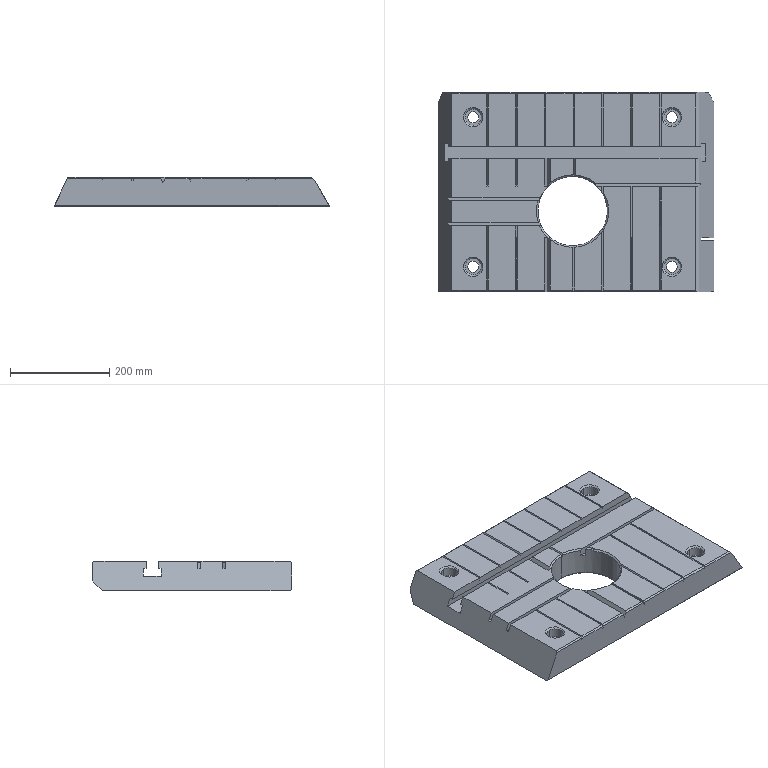Component | SolidWorks | WorkbenchPanel-1 | 1 solid | 158 faces | volume 10820367 mm3 | plane 122 | cone 18 | cylinder 18 | commonest cylinder face diameters 33 x8 22 x8 140 x2